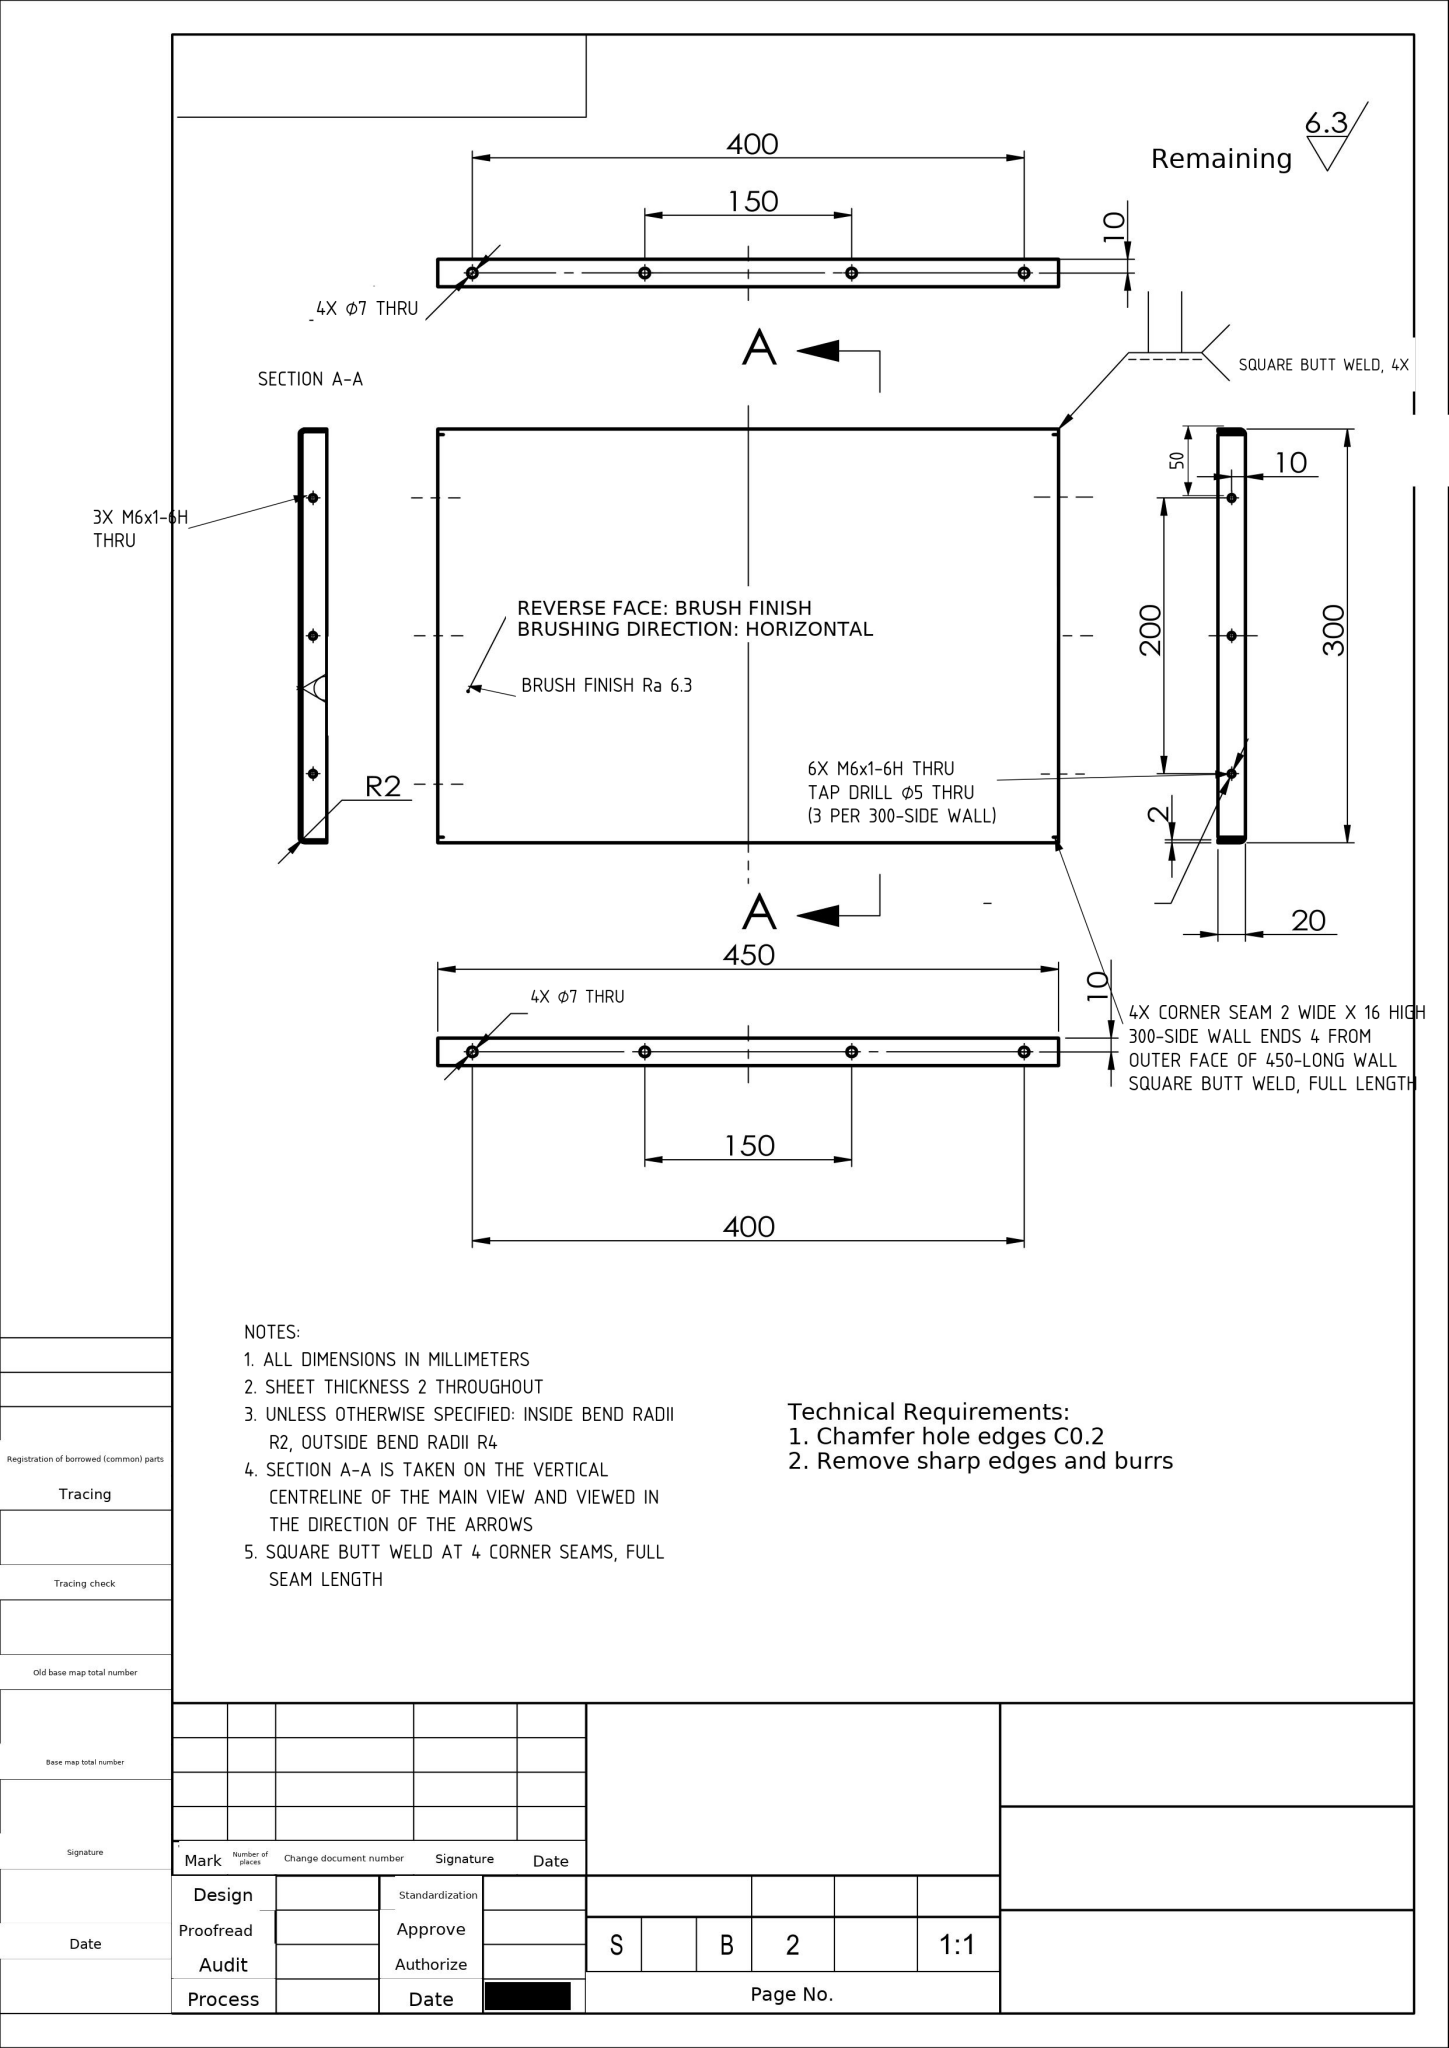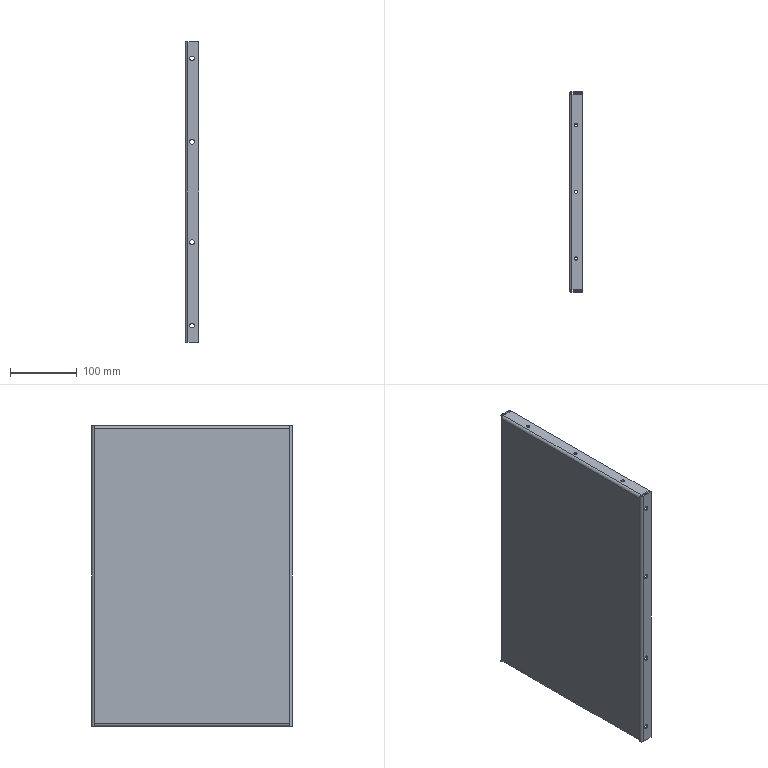Part | NX | mm | 1 solid | 70 faces | box 20 x 300 x 450 mm | volume 318751 mm3 | cylinder 36 | plane 34 | commonest cylinder face diameters 7 x16 5 x12 4 x4 8 x4